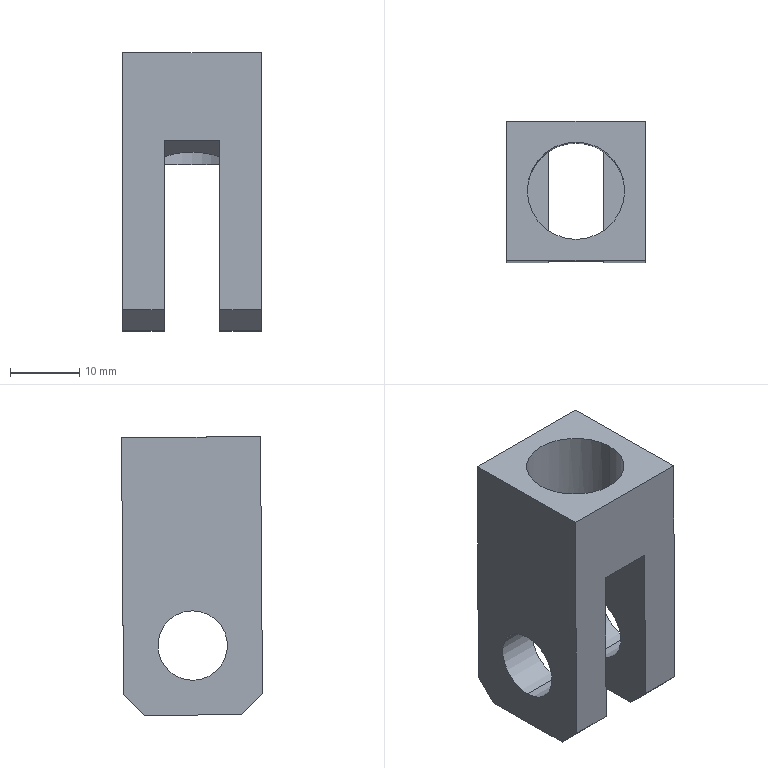Component | SolidWorks | OT-0100-008(LiveHinge)-1 | 1 solid | 23 faces | box 20 x 20.3 x 40.14 mm | volume 8582 mm3 | plane 17 | cylinder 6 | commonest cylinder face diameters 10 x4 14 x2 | material Plain Carbon Steel
build123d program:
from build123d import *

# Parameters (mm, degrees)
SKETCH1_W                  = 40
SKETCH1_H                  = 20
BOSS_EXTRUDE1_DEPTH        = 10
CUT_EXTRUDE1_REACH         = 47.826
SKETCH2_W                  = 24
SKETCH2_H                  = 8
M14X1_5_TAPPED_HOLE1_D     = 14
M14X1_5_TAPPED_HOLE1_DEPTH = 16
SKETCH5_R                  = 5
CUT_EXTRUDE2_DEPTH         = 46.826
CHAMFER1_SIZE              = 3
LUG_CLEARANCE_RELIEF_DEPTH = 4


with BuildPart() as part:
    # Sketch1 → Boss-Extrude1 (new, symmetric)
    with BuildSketch(Plane(origin=(0, 0, 0), x_dir=(1, 0, 0), z_dir=(0, 1, 0))):
        with Locations((20, 0)):
            Rectangle(SKETCH1_W, SKETCH1_H)
    extrude(amount=BOSS_EXTRUDE1_DEPTH, both=True)

    # Sketch2 → Cut-Extrude1 (cut, up to next)
    with BuildSketch(Plane(origin=(0, 10, 0), x_dir=(1, 0, 0), z_dir=(0, 1, 0)), mode=Mode.PRIVATE) as cut_extrude1_sk1:
        with Locations((12, 0)):
            Rectangle(SKETCH2_W, SKETCH2_H)
    cut_extrude1_tool1 = extrude(cut_extrude1_sk1.sketch, amount=-CUT_EXTRUDE1_REACH, mode=Mode.PRIVATE) & part.part
    add(cut_extrude1_tool1.solids().sort_by_distance((12, 10, 0))[0], mode=Mode.SUBTRACT)

    # M14x1.5 Tapped Hole1
    with Locations(Plane(origin=(40, 0, 0), x_dir=(0, 0, -1), z_dir=(1, 0, 0))):
        with Locations((0, 0)):
            Hole(M14X1_5_TAPPED_HOLE1_D / 2, depth=M14X1_5_TAPPED_HOLE1_DEPTH)

    # Sketch5 → Cut-Extrude2 (cut, through all)
    with BuildSketch(Plane.XY.offset(10)):
        with Locations((10, 0)):
            Circle(SKETCH5_R)
    extrude(amount=-CUT_EXTRUDE2_DEPTH, mode=Mode.SUBTRACT)

    # Chamfer1
    chamfer1_edges = [part.edges().sort_by_distance(p)[0] for p in [
        (0, -10, 7),
        (0, 10, 7),
        (0, 10, -7),
        (0, -10, -7),
    ]]
    chamfer(chamfer1_edges, length=CHAMFER1_SIZE)

    # Lug-clearance relief sketch → Lug-clearance relief (cut, symmetric)
    with BuildSketch(Plane.XY):
        Polygon((28.386, -12), (22, -0.1392), (22, -12), align=None)
    extrude(amount=LUG_CLEARANCE_RELIEF_DEPTH, both=True, mode=Mode.SUBTRACT)


solid = part.part

# Placed as in the assembly
solid = solid.moved(Location((200, 104.892, -36.996), (-0.4615, -90, 0)))
STEP:
#1=COLOUR_RGB('',0.7922,0.8196,0.9333);
#2=FILL_AREA_STYLE_COLOUR('',#1);
#3=FILL_AREA_STYLE('',(#2));
#4=SURFACE_STYLE_FILL_AREA(#3);
#5=SURFACE_SIDE_STYLE('',(#4));
#6=SURFACE_STYLE_USAGE(.BOTH.,#5);
#7=PRESENTATION_STYLE_ASSIGNMENT((#6));
#8=CARTESIAN_POINT('',(8.268,4.131,-1.26));
#9=VERTEX_POINT('',#8);
#10=CARTESIAN_POINT('',(8.268,4.134,-0.866));
#11=VERTEX_POINT('',#10);
#12=CARTESIAN_POINT('',(8.268,4.133,-1.063));
#13=DIRECTION('',(-1.,0.,-0.));
#14=DIRECTION('',(0.,0.008055,1.));
#15=AXIS2_PLACEMENT_3D('',#12,#13,#14);
#16=CIRCLE('',#15,0.1969);
#17=EDGE_CURVE('',#9,#11,#16,.T.);
#18=ORIENTED_EDGE('',*,*,#17,.F.);
#19=CARTESIAN_POINT('',(8.031,4.131,-1.26));
#20=VERTEX_POINT('',#19);
#21=CARTESIAN_POINT('',(8.268,4.131,-1.26));
#22=DIRECTION('',(-1.,0.,-0.));
#23=VECTOR('',#22,39.37);
#24=LINE('',#21,#23);
#25=EDGE_CURVE('',#9,#20,#24,.T.);
#26=ORIENTED_EDGE('',*,*,#25,.T.);
#27=CARTESIAN_POINT('',(8.031,4.134,-0.866));
#28=VERTEX_POINT('',#27);
#29=CARTESIAN_POINT('',(8.031,4.133,-1.063));
#30=DIRECTION('',(1.,-0.,0.));
#31=DIRECTION('',(0.,-0.008055,-1.));
#32=AXIS2_PLACEMENT_3D('',#29,#30,#31);
#33=CIRCLE('',#32,0.1969);
#34=EDGE_CURVE('',#28,#20,#33,.T.);
#35=ORIENTED_EDGE('',*,*,#34,.F.);
#36=CARTESIAN_POINT('',(8.268,4.134,-0.866));
#37=DIRECTION('',(-1.,0.,-0.));
#38=VECTOR('',#37,39.37);
#39=LINE('',#36,#38);
#40=EDGE_CURVE('',#11,#28,#39,.T.);
#41=ORIENTED_EDGE('',*,*,#40,.F.);
#42=EDGE_LOOP('',(#18,#26,#35,#41));
#43=FACE_OUTER_BOUND('',#42,.T.);
#44=CARTESIAN_POINT('',(8.268,4.133,-1.063));
#45=DIRECTION('',(-1.,0.,-0.));
#46=DIRECTION('',(0.,0.008055,1.));
#47=AXIS2_PLACEMENT_3D('',#44,#45,#46);
#48=CYLINDRICAL_SURFACE('',#47,0.1969);
#49=ADVANCED_FACE('',(#43),#48,.F.);
#50=CARTESIAN_POINT('',(7.717,4.131,-1.26));
#51=VERTEX_POINT('',#50);
#52=CARTESIAN_POINT('',(7.717,4.134,-0.866));
#53=VERTEX_POINT('',#52);
#54=CARTESIAN_POINT('',(7.717,4.133,-1.063));
#55=DIRECTION('',(-1.,0.,-0.));
#56=DIRECTION('',(0.,0.008055,1.));
#57=AXIS2_PLACEMENT_3D('',#54,#55,#56);
#58=CIRCLE('',#57,0.1969);
#59=EDGE_CURVE('',#51,#53,#58,.T.);
#60=ORIENTED_EDGE('',*,*,#59,.F.);
#61=CARTESIAN_POINT('',(7.48,4.131,-1.26));
#62=VERTEX_POINT('',#61);
#63=CARTESIAN_POINT('',(8.268,4.131,-1.26));
#64=DIRECTION('',(-1.,0.,-0.));
#65=VECTOR('',#64,39.37);
#66=LINE('',#63,#65);
#67=EDGE_CURVE('',#51,#62,#66,.T.);
#68=ORIENTED_EDGE('',*,*,#67,.T.);
#69=CARTESIAN_POINT('',(7.48,4.134,-0.866));
#70=VERTEX_POINT('',#69);
#71=CARTESIAN_POINT('',(7.48,4.133,-1.063));
#72=DIRECTION('',(-1.,0.,-0.));
#73=DIRECTION('',(0.,0.008055,1.));
#74=AXIS2_PLACEMENT_3D('',#71,#72,#73);
#75=CIRCLE('',#74,0.1969);
#76=EDGE_CURVE('',#62,#70,#75,.T.);
#77=ORIENTED_EDGE('',*,*,#76,.T.);
#78=CARTESIAN_POINT('',(8.268,4.134,-0.866));
#79=DIRECTION('',(-1.,0.,-0.));
#80=VECTOR('',#79,39.37);
#81=LINE('',#78,#80);
#82=EDGE_CURVE('',#53,#70,#81,.T.);
#83=ORIENTED_EDGE('',*,*,#82,.F.);
#84=EDGE_LOOP('',(#60,#68,#77,#83));
#85=FACE_OUTER_BOUND('',#84,.T.);
#86=CARTESIAN_POINT('',(8.268,4.133,-1.063));
#87=DIRECTION('',(-1.,0.,-0.));
#88=DIRECTION('',(0.,0.008055,1.));
#89=AXIS2_PLACEMENT_3D('',#86,#87,#88);
#90=CYLINDRICAL_SURFACE('',#89,0.1969);
#91=ADVANCED_FACE('',(#85),#90,.F.);
#92=CARTESIAN_POINT('',(7.717,3.911,-0.5098));
#93=VERTEX_POINT('',#92);
#94=CARTESIAN_POINT('',(7.598,4.137,-0.5117));
#95=VERTEX_POINT('',#94);
#96=CARTESIAN_POINT('',(7.874,4.137,-0.5117));
#97=DIRECTION('',(0.,-0.008055,-1.));
#98=DIRECTION('',(1.,0.,0.));
#99=AXIS2_PLACEMENT_3D('',#96,#97,#98);
#100=CIRCLE('',#99,0.2756);
#101=EDGE_CURVE('',#93,#95,#100,.T.);
#102=ORIENTED_EDGE('',*,*,#101,.T.);
#103=CARTESIAN_POINT('',(7.598,4.142,0.1182));
#104=VERTEX_POINT('',#103);
#105=CARTESIAN_POINT('',(7.598,4.142,0.1182));
#106=DIRECTION('',(-0.,0.008055,1.));
#107=VECTOR('',#106,39.37);
#108=LINE('',#105,#107);
#109=EDGE_CURVE('',#95,#104,#108,.T.);
#110=ORIENTED_EDGE('',*,*,#109,.T.);
#111=CARTESIAN_POINT('',(8.15,4.142,0.1182));
#112=VERTEX_POINT('',#111);
#113=CARTESIAN_POINT('',(7.874,4.142,0.1182));
#114=DIRECTION('',(-0.,0.008055,1.));
#115=DIRECTION('',(1.,0.,0.));
#116=AXIS2_PLACEMENT_3D('',#113,#114,#115);
#117=CIRCLE('',#116,0.2756);
#118=EDGE_CURVE('',#104,#112,#117,.T.);
#119=ORIENTED_EDGE('',*,*,#118,.T.);
#120=CARTESIAN_POINT('',(8.15,4.137,-0.5117));
#121=VERTEX_POINT('',#120);
#122=CARTESIAN_POINT('',(8.15,4.142,0.1182));
#123=DIRECTION('',(-0.,0.008055,1.));
#124=VECTOR('',#123,39.37);
#125=LINE('',#122,#124);
#126=EDGE_CURVE('',#121,#112,#125,.T.);
#127=ORIENTED_EDGE('',*,*,#126,.F.);
#128=CARTESIAN_POINT('',(8.031,3.911,-0.5098));
#129=VERTEX_POINT('',#128);
#130=CARTESIAN_POINT('',(7.874,4.137,-0.5117));
#131=DIRECTION('',(0.,-0.008055,-1.));
#132=DIRECTION('',(1.,0.,0.));
#133=AXIS2_PLACEMENT_3D('',#130,#131,#132);
#134=CIRCLE('',#133,0.2756);
#135=EDGE_CURVE('',#121,#129,#134,.T.);
#136=ORIENTED_EDGE('',*,*,#135,.T.);
#137=CARTESIAN_POINT('',(8.031,3.911,-0.4698));
#138=VERTEX_POINT('',#137);
#139=CARTESIAN_POINT('',(8.031,3.916,0.1201));
#140=DIRECTION('',(-0.,0.008055,1.));
#141=VECTOR('',#140,39.37);
#142=LINE('',#139,#141);
#143=EDGE_CURVE('',#129,#138,#142,.T.);
#144=ORIENTED_EDGE('',*,*,#143,.T.);
#145=CARTESIAN_POINT('',(7.717,3.911,-0.4698));
#146=VERTEX_POINT('',#145);
#147=CARTESIAN_POINT('',(8.031,3.911,-0.4698));
#148=CARTESIAN_POINT('',(7.934,3.844,-0.4325));
#149=CARTESIAN_POINT('',(7.814,3.844,-0.4325));
#150=CARTESIAN_POINT('',(7.717,3.911,-0.4698));
#151=(BOUNDED_CURVE()B_SPLINE_CURVE(3,(#147,#148,#149,#150),.UNSPECIFIED.,.F.,.F.)B_SPLINE_CURVE_WITH_KNOTS((4,4),(5.675,6.891),.UNSPECIFIED.)CURVE()GEOMETRIC_REPRESENTATION_ITEM()RATIONAL_B_SPLINE_CURVE((1.,0.8804,0.8804,1.))REPRESENTATION_ITEM(''));
#152=EDGE_CURVE('',#138,#146,#151,.T.);
#153=ORIENTED_EDGE('',*,*,#152,.T.);
#154=CARTESIAN_POINT('',(7.717,3.916,0.1201));
#155=DIRECTION('',(-0.,0.008055,1.));
#156=VECTOR('',#155,39.37);
#157=LINE('',#154,#156);
#158=EDGE_CURVE('',#93,#146,#157,.T.);
#159=ORIENTED_EDGE('',*,*,#158,.F.);
#160=EDGE_LOOP('',(#102,#110,#119,#127,#136,#144,#153,#159));
#161=FACE_OUTER_BOUND('',#160,.T.);
#162=CARTESIAN_POINT('',(7.874,4.142,0.1182));
#163=DIRECTION('',(-0.,0.008055,1.));
#164=DIRECTION('',(1.,0.,0.));
#165=AXIS2_PLACEMENT_3D('',#162,#163,#164);
#166=CYLINDRICAL_SURFACE('',#165,0.2756);
#167=ADVANCED_FACE('',(#161),#166,.F.);
#168=CARTESIAN_POINT('',(8.031,4.363,-0.5135));
#169=VERTEX_POINT('',#168);
#170=CARTESIAN_POINT('',(8.031,4.531,-0.5148));
#171=VERTEX_POINT('',#170);
#172=CARTESIAN_POINT('',(8.031,3.744,-0.5085));
#173=DIRECTION('',(0.,1.,-0.008055));
#174=VECTOR('',#173,39.37);
#175=LINE('',#172,#174);
#176=EDGE_CURVE('',#169,#171,#175,.T.);
#177=ORIENTED_EDGE('',*,*,#176,.F.);
#178=CARTESIAN_POINT('',(7.717,4.363,-0.5135));
#179=VERTEX_POINT('',#178);
#180=CARTESIAN_POINT('',(7.874,4.137,-0.5117));
#181=DIRECTION('',(-0.,0.008055,1.));
#182=DIRECTION('',(1.,0.,0.));
#183=AXIS2_PLACEMENT_3D('',#180,#181,#182);
#184=CIRCLE('',#183,0.2756);
#185=EDGE_CURVE('',#169,#179,#184,.T.);
#186=ORIENTED_EDGE('',*,*,#185,.T.);
#187=CARTESIAN_POINT('',(7.717,4.531,-0.5148));
#188=VERTEX_POINT('',#187);
#189=CARTESIAN_POINT('',(7.717,3.744,-0.5085));
#190=DIRECTION('',(0.,1.,-0.008055));
#191=VECTOR('',#190,39.37);
#192=LINE('',#189,#191);
#193=EDGE_CURVE('',#179,#188,#192,.T.);
#194=ORIENTED_EDGE('',*,*,#193,.T.);
#195=CARTESIAN_POINT('',(7.717,4.531,-0.5148));
#196=DIRECTION('',(1.,-0.,0.));
#197=VECTOR('',#196,39.37);
#198=LINE('',#195,#197);
#199=EDGE_CURVE('',#188,#171,#198,.T.);
#200=ORIENTED_EDGE('',*,*,#199,.T.);
#201=EDGE_LOOP('',(#177,#186,#194,#200));
#202=FACE_OUTER_BOUND('',#201,.T.);
#203=CARTESIAN_POINT('',(7.717,3.744,-0.5085));
#204=DIRECTION('',(-0.,0.008055,1.));
#205=DIRECTION('',(1.,-0.,0.));
#206=AXIS2_PLACEMENT_3D('',#203,#204,#205);
#207=PLANE('',#206);
#208=ADVANCED_FACE('',(#202),#207,.F.);
#209=CARTESIAN_POINT('',(8.268,4.405,-1.459));
#210=VERTEX_POINT('',#209);
#211=CARTESIAN_POINT('',(8.268,3.854,-1.454));
#212=VERTEX_POINT('',#211);
#213=CARTESIAN_POINT('',(8.268,4.523,-1.46));
#214=DIRECTION('',(-0.,-1.,0.008055));
#215=VECTOR('',#214,39.37);
#216=LINE('',#213,#215);
#217=EDGE_CURVE('',#210,#212,#216,.T.);
#218=ORIENTED_EDGE('',*,*,#217,.T.);
#219=CARTESIAN_POINT('',(8.031,3.854,-1.454));
#220=VERTEX_POINT('',#219);
#221=CARTESIAN_POINT('',(8.031,3.854,-1.454));
#222=DIRECTION('',(-1.,0.,-0.));
#223=VECTOR('',#222,39.37);
#224=LINE('',#221,#223);
#225=EDGE_CURVE('',#212,#220,#224,.T.);
#226=ORIENTED_EDGE('',*,*,#225,.T.);
#227=CARTESIAN_POINT('',(8.031,4.405,-1.459));
#228=VERTEX_POINT('',#227);
#229=CARTESIAN_POINT('',(8.031,3.736,-1.453));
#230=DIRECTION('',(0.,1.,-0.008055));
#231=VECTOR('',#230,39.37);
#232=LINE('',#229,#231);
#233=EDGE_CURVE('',#220,#228,#232,.T.);
#234=ORIENTED_EDGE('',*,*,#233,.T.);
#235=CARTESIAN_POINT('',(7.48,4.405,-1.459));
#236=DIRECTION('',(1.,-0.,0.));
#237=VECTOR('',#236,39.37);
#238=LINE('',#235,#237);
#239=EDGE_CURVE('',#228,#210,#238,.T.);
#240=ORIENTED_EDGE('',*,*,#239,.T.);
#241=EDGE_LOOP('',(#218,#226,#234,#240));
#242=FACE_OUTER_BOUND('',#241,.T.);
#243=CARTESIAN_POINT('',(7.48,4.523,-1.46));
#244=DIRECTION('',(-0.,0.008055,1.));
#245=DIRECTION('',(1.,-0.,0.));
#246=AXIS2_PLACEMENT_3D('',#243,#244,#245);
#247=PLANE('',#246);
#248=ADVANCED_FACE('',(#242),#247,.F.);
#249=CARTESIAN_POINT('',(7.717,3.854,-1.454));
#250=VERTEX_POINT('',#249);
#251=CARTESIAN_POINT('',(7.717,4.405,-1.459));
#252=VERTEX_POINT('',#251);
#253=CARTESIAN_POINT('',(7.717,3.736,-1.453));
#254=DIRECTION('',(0.,1.,-0.008055));
#255=VECTOR('',#254,39.37);
#256=LINE('',#253,#255);
#257=EDGE_CURVE('',#250,#252,#256,.T.);
#258=ORIENTED_EDGE('',*,*,#257,.F.);
#259=CARTESIAN_POINT('',(7.48,3.854,-1.454));
#260=VERTEX_POINT('',#259);
#261=CARTESIAN_POINT('',(7.48,3.854,-1.454));
#262=DIRECTION('',(-1.,0.,-0.));
#263=VECTOR('',#262,39.37);
#264=LINE('',#261,#263);
#265=EDGE_CURVE('',#250,#260,#264,.T.);
#266=ORIENTED_EDGE('',*,*,#265,.T.);
#267=CARTESIAN_POINT('',(7.48,4.405,-1.459));
#268=VERTEX_POINT('',#267);
#269=CARTESIAN_POINT('',(7.48,4.523,-1.46));
#270=DIRECTION('',(-0.,-1.,0.008055));
#271=VECTOR('',#270,39.37);
#272=LINE('',#269,#271);
#273=EDGE_CURVE('',#268,#260,#272,.T.);
#274=ORIENTED_EDGE('',*,*,#273,.F.);
#275=CARTESIAN_POINT('',(7.48,4.405,-1.459));
#276=DIRECTION('',(1.,-0.,0.));
#277=VECTOR('',#276,39.37);
#278=LINE('',#275,#277);
#279=EDGE_CURVE('',#268,#252,#278,.T.);
#280=ORIENTED_EDGE('',*,*,#279,.T.);
#281=EDGE_LOOP('',(#258,#266,#274,#280));
#282=FACE_OUTER_BOUND('',#281,.T.);
#283=CARTESIAN_POINT('',(7.48,4.523,-1.46));
#284=DIRECTION('',(-0.,0.008055,1.));
#285=DIRECTION('',(1.,-0.,0.));
#286=AXIS2_PLACEMENT_3D('',#283,#284,#285);
#287=PLANE('',#286);
#288=ADVANCED_FACE('',(#282),#287,.F.);
#289=CARTESIAN_POINT('',(7.48,4.133,-1.063));
#290=DIRECTION('',(-1.,0.,-0.));
#291=DIRECTION('',(0.,0.008055,1.));
#292=AXIS2_PLACEMENT_3D('',#289,#290,#291);
#293=CIRCLE('',#292,0.1969);
#294=EDGE_CURVE('',#70,#62,#293,.T.);
#295=ORIENTED_EDGE('',*,*,#294,.F.);
#296=ORIENTED_EDGE('',*,*,#76,.F.);
#297=EDGE_LOOP('',(#295,#296));
#298=FACE_BOUND('',#297,.T.);
#299=ORIENTED_EDGE('',*,*,#273,.T.);
#300=CARTESIAN_POINT('',(7.48,3.737,-1.335));
#301=VERTEX_POINT('',#300);
#302=CARTESIAN_POINT('',(7.48,3.854,-1.454));
#303=DIRECTION('',(-0.,-0.7014,0.7128));
#304=VECTOR('',#303,39.37);
#305=LINE('',#302,#304);
#306=EDGE_CURVE('',#260,#301,#305,.T.);
#307=ORIENTED_EDGE('',*,*,#306,.T.);
#308=CARTESIAN_POINT('',(7.48,3.749,0.1214));
#309=VERTEX_POINT('',#308);
#310=CARTESIAN_POINT('',(7.48,3.736,-1.453));
#311=DIRECTION('',(-0.,0.008055,1.));
#312=VECTOR('',#311,39.37);
#313=LINE('',#310,#312);
#314=EDGE_CURVE('',#301,#309,#313,.T.);
#315=ORIENTED_EDGE('',*,*,#314,.T.);
#316=CARTESIAN_POINT('',(7.48,4.536,0.1151));
#317=VERTEX_POINT('',#316);
#318=CARTESIAN_POINT('',(7.48,4.536,0.1151));
#319=DIRECTION('',(-0.,-1.,0.008055));
#320=VECTOR('',#319,39.37);
#321=LINE('',#318,#320);
#322=EDGE_CURVE('',#317,#309,#321,.T.);
#323=ORIENTED_EDGE('',*,*,#322,.F.);
#324=CARTESIAN_POINT('',(7.48,4.524,-1.342));
#325=VERTEX_POINT('',#324);
#326=CARTESIAN_POINT('',(7.48,4.523,-1.46));
#327=DIRECTION('',(-0.,0.008055,1.));
#328=VECTOR('',#327,39.37);
#329=LINE('',#326,#328);
#330=EDGE_CURVE('',#325,#317,#329,.T.);
#331=ORIENTED_EDGE('',*,*,#330,.F.);
#332=CARTESIAN_POINT('',(7.48,4.524,-1.342));
#333=DIRECTION('',(-0.,-0.7128,-0.7014));
#334=VECTOR('',#333,39.37);
#335=LINE('',#332,#334);
#336=EDGE_CURVE('',#325,#268,#335,.T.);
#337=ORIENTED_EDGE('',*,*,#336,.T.);
#338=EDGE_LOOP('',(#299,#307,#315,#323,#331,#337));
#339=FACE_OUTER_BOUND('',#338,.T.);
#340=CARTESIAN_POINT('',(7.48,4.523,-1.46));
#341=DIRECTION('',(1.,-0.,0.));
#342=DIRECTION('',(0.,-0.008055,-1.));
#343=AXIS2_PLACEMENT_3D('',#340,#341,#342);
#344=PLANE('',#343);
#345=ADVANCED_FACE('',(#298,#339),#344,.F.);
#346=CARTESIAN_POINT('',(7.874,4.142,0.1182));
#347=DIRECTION('',(-0.,0.008055,1.));
#348=DIRECTION('',(1.,0.,0.));
#349=AXIS2_PLACEMENT_3D('',#346,#347,#348);
#350=CIRCLE('',#349,0.2756);
#351=EDGE_CURVE('',#112,#104,#350,.T.);
#352=ORIENTED_EDGE('',*,*,#351,.F.);
#353=ORIENTED_EDGE('',*,*,#118,.F.);
#354=EDGE_LOOP('',(#352,#353));
#355=FACE_BOUND('',#354,.T.);
#356=CARTESIAN_POINT('',(8.268,3.749,0.1214));
#357=VERTEX_POINT('',#356);
#358=CARTESIAN_POINT('',(7.48,3.749,0.1214));
#359=DIRECTION('',(1.,-0.,0.));
#360=VECTOR('',#359,39.37);
#361=LINE('',#358,#360);
#362=EDGE_CURVE('',#309,#357,#361,.T.);
#363=ORIENTED_EDGE('',*,*,#362,.T.);
#364=CARTESIAN_POINT('',(8.268,4.536,0.1151));
#365=VERTEX_POINT('',#364);
#366=CARTESIAN_POINT('',(8.268,4.536,0.1151));
#367=DIRECTION('',(-0.,-1.,0.008055));
#368=VECTOR('',#367,39.37);
#369=LINE('',#366,#368);
#370=EDGE_CURVE('',#365,#357,#369,.T.);
#371=ORIENTED_EDGE('',*,*,#370,.F.);
#372=CARTESIAN_POINT('',(7.48,4.536,0.1151));
#373=DIRECTION('',(1.,-0.,0.));
#374=VECTOR('',#373,39.37);
#375=LINE('',#372,#374);
#376=EDGE_CURVE('',#317,#365,#375,.T.);
#377=ORIENTED_EDGE('',*,*,#376,.F.);
#378=ORIENTED_EDGE('',*,*,#322,.T.);
#379=EDGE_LOOP('',(#363,#371,#377,#378));
#380=FACE_OUTER_BOUND('',#379,.T.);
#381=CARTESIAN_POINT('',(7.48,4.536,0.1151));
#382=DIRECTION('',(0.,-0.008055,-1.));
#383=DIRECTION('',(-1.,0.,-0.));
#384=AXIS2_PLACEMENT_3D('',#381,#382,#383);
#385=PLANE('',#384);
#386=ADVANCED_FACE('',(#355,#380),#385,.F.);
#387=CARTESIAN_POINT('',(8.268,4.133,-1.063));
#388=DIRECTION('',(-1.,0.,-0.));
#389=DIRECTION('',(0.,0.008055,1.));
#390=AXIS2_PLACEMENT_3D('',#387,#388,#389);
#391=CIRCLE('',#390,0.1969);
#392=EDGE_CURVE('',#11,#9,#391,.T.);
#393=ORIENTED_EDGE('',*,*,#392,.T.);
#394=ORIENTED_EDGE('',*,*,#17,.T.);
#395=EDGE_LOOP('',(#393,#394));
#396=FACE_BOUND('',#395,.T.);
#397=CARTESIAN_POINT('',(8.268,3.737,-1.335));
#398=VERTEX_POINT('',#397);
#399=CARTESIAN_POINT('',(8.268,3.736,-1.453));
#400=DIRECTION('',(-0.,-0.008055,-1.));
#401=VECTOR('',#400,39.37);
#402=LINE('',#399,#401);
#403=EDGE_CURVE('',#357,#398,#402,.T.);
#404=ORIENTED_EDGE('',*,*,#403,.T.);
#405=CARTESIAN_POINT('',(8.268,3.854,-1.454));
#406=DIRECTION('',(-0.,0.7014,-0.7128));
#407=VECTOR('',#406,39.37);
#408=LINE('',#405,#407);
#409=EDGE_CURVE('',#398,#212,#408,.T.);
#410=ORIENTED_EDGE('',*,*,#409,.T.);
#411=ORIENTED_EDGE('',*,*,#217,.F.);
#412=CARTESIAN_POINT('',(8.268,4.524,-1.342));
#413=VERTEX_POINT('',#412);
#414=CARTESIAN_POINT('',(8.268,4.524,-1.342));
#415=DIRECTION('',(0.,0.7128,0.7014));
#416=VECTOR('',#415,39.37);
#417=LINE('',#414,#416);
#418=EDGE_CURVE('',#210,#413,#417,.T.);
#419=ORIENTED_EDGE('',*,*,#418,.T.);
#420=CARTESIAN_POINT('',(8.268,4.523,-1.46));
#421=DIRECTION('',(-0.,-0.008055,-1.));
#422=VECTOR('',#421,39.37);
#423=LINE('',#420,#422);
#424=EDGE_CURVE('',#365,#413,#423,.T.);
#425=ORIENTED_EDGE('',*,*,#424,.F.);
#426=ORIENTED_EDGE('',*,*,#370,.T.);
#427=EDGE_LOOP('',(#404,#410,#411,#419,#425,#426));
#428=FACE_OUTER_BOUND('',#427,.T.);
#429=CARTESIAN_POINT('',(8.268,4.523,-1.46));
#430=DIRECTION('',(-1.,0.,0.));
#431=DIRECTION('',(0.,0.008055,1.));
#432=AXIS2_PLACEMENT_3D('',#429,#430,#431);
#433=PLANE('',#432);
#434=ADVANCED_FACE('',(#396,#428),#433,.F.);
#435=ORIENTED_EDGE('',*,*,#424,.T.);
#436=CARTESIAN_POINT('',(8.031,4.524,-1.342));
#437=VERTEX_POINT('',#436);
#438=CARTESIAN_POINT('',(7.874,4.524,-1.342));
#439=DIRECTION('',(-1.,0.,-0.));
#440=VECTOR('',#439,39.37);
#441=LINE('',#438,#440);
#442=EDGE_CURVE('',#413,#437,#441,.T.);
#443=ORIENTED_EDGE('',*,*,#442,.T.);
#444=CARTESIAN_POINT('',(8.031,4.523,-1.46));
#445=DIRECTION('',(0.,-0.008055,-1.));
#446=VECTOR('',#445,39.37);
#447=LINE('',#444,#446);
#448=EDGE_CURVE('',#171,#437,#447,.T.);
#449=ORIENTED_EDGE('',*,*,#448,.F.);
#450=ORIENTED_EDGE('',*,*,#199,.F.);
#451=CARTESIAN_POINT('',(7.717,4.524,-1.342));
#452=VERTEX_POINT('',#451);
#453=CARTESIAN_POINT('',(7.717,4.523,-1.46));
#454=DIRECTION('',(-0.,0.008055,1.));
#455=VECTOR('',#454,39.37);
#456=LINE('',#453,#455);
#457=EDGE_CURVE('',#452,#188,#456,.T.);
#458=ORIENTED_EDGE('',*,*,#457,.F.);
#459=CARTESIAN_POINT('',(7.874,4.524,-1.342));
#460=DIRECTION('',(-1.,0.,-0.));
#461=VECTOR('',#460,39.37);
#462=LINE('',#459,#461);
#463=EDGE_CURVE('',#452,#325,#462,.T.);
#464=ORIENTED_EDGE('',*,*,#463,.T.);
#465=ORIENTED_EDGE('',*,*,#330,.T.);
#466=ORIENTED_EDGE('',*,*,#376,.T.);
#467=EDGE_LOOP('',(#435,#443,#449,#450,#458,#464,#465,#466));
#468=FACE_OUTER_BOUND('',#467,.T.);
#469=CARTESIAN_POINT('',(7.874,4.523,-1.46));
#470=DIRECTION('',(-0.,-1.,0.008055));
#471=DIRECTION('',(1.,-0.,0.));
#472=AXIS2_PLACEMENT_3D('',#469,#470,#471);
#473=PLANE('',#472);
#474=ADVANCED_FACE('',(#468),#473,.F.);
#475=CARTESIAN_POINT('',(8.031,3.745,-0.3782));
#476=VERTEX_POINT('',#475);
#477=CARTESIAN_POINT('',(7.717,3.745,-0.3782));
#478=VERTEX_POINT('',#477);
#479=CARTESIAN_POINT('',(7.874,3.745,-0.3782));
#480=DIRECTION('',(-1.,0.,-0.));
#481=VECTOR('',#480,39.37);
#482=LINE('',#479,#481);
#483=EDGE_CURVE('',#476,#478,#482,.T.);
#484=ORIENTED_EDGE('',*,*,#483,.F.);
#485=CARTESIAN_POINT('',(8.031,3.737,-1.335));
#486=VERTEX_POINT('',#485);
#487=CARTESIAN_POINT('',(8.031,3.736,-1.453));
#488=DIRECTION('',(0.,-0.008055,-1.));
#489=VECTOR('',#488,39.37);
#490=LINE('',#487,#489);
#491=EDGE_CURVE('',#476,#486,#490,.T.);
#492=ORIENTED_EDGE('',*,*,#491,.T.);
#493=CARTESIAN_POINT('',(8.268,3.737,-1.335));
#494=DIRECTION('',(1.,-0.,0.));
#495=VECTOR('',#494,39.37);
#496=LINE('',#493,#495);
#497=EDGE_CURVE('',#486,#398,#496,.T.);
#498=ORIENTED_EDGE('',*,*,#497,.T.);
#499=ORIENTED_EDGE('',*,*,#403,.F.);
#500=ORIENTED_EDGE('',*,*,#362,.F.);
#501=ORIENTED_EDGE('',*,*,#314,.F.);
#502=CARTESIAN_POINT('',(7.717,3.737,-1.335));
#503=VERTEX_POINT('',#502);
#504=CARTESIAN_POINT('',(7.717,3.737,-1.335));
#505=DIRECTION('',(1.,-0.,0.));
#506=VECTOR('',#505,39.37);
#507=LINE('',#504,#506);
#508=EDGE_CURVE('',#301,#503,#507,.T.);
#509=ORIENTED_EDGE('',*,*,#508,.T.);
#510=CARTESIAN_POINT('',(7.717,3.736,-1.453));
#511=DIRECTION('',(-0.,0.008055,1.));
#512=VECTOR('',#511,39.37);
#513=LINE('',#510,#512);
#514=EDGE_CURVE('',#503,#478,#513,.T.);
#515=ORIENTED_EDGE('',*,*,#514,.T.);
#516=EDGE_LOOP('',(#484,#492,#498,#499,#500,#501,#509,#515));
#517=FACE_OUTER_BOUND('',#516,.T.);
#518=CARTESIAN_POINT('',(7.874,3.736,-1.453));
#519=DIRECTION('',(-0.,-1.,0.008055));
#520=DIRECTION('',(1.,-0.,0.));
#521=AXIS2_PLACEMENT_3D('',#518,#519,#520);
#522=PLANE('',#521);
#523=ADVANCED_FACE('',(#517),#522,.T.);
#524=CARTESIAN_POINT('',(8.031,3.854,-1.454));
#525=DIRECTION('',(-0.,-0.7014,0.7128));
#526=VECTOR('',#525,39.37);
#527=LINE('',#524,#526);
#528=EDGE_CURVE('',#220,#486,#527,.T.);
#529=ORIENTED_EDGE('',*,*,#528,.T.);
#530=ORIENTED_EDGE('',*,*,#491,.F.);
#531=CARTESIAN_POINT('',(8.031,3.666,-0.3352));
#532=DIRECTION('',(0.,0.8767,-0.4811));
#533=VECTOR('',#532,39.37);
#534=LINE('',#531,#533);
#535=EDGE_CURVE('',#476,#138,#534,.T.);
#536=ORIENTED_EDGE('',*,*,#535,.T.);
#537=ORIENTED_EDGE('',*,*,#143,.F.);
#538=CARTESIAN_POINT('',(8.031,3.744,-0.5085));
#539=DIRECTION('',(0.,1.,-0.008055));
#540=VECTOR('',#539,39.37);
#541=LINE('',#538,#540);
#542=EDGE_CURVE('',#129,#169,#541,.T.);
#543=ORIENTED_EDGE('',*,*,#542,.T.);
#544=ORIENTED_EDGE('',*,*,#176,.T.);
#545=ORIENTED_EDGE('',*,*,#448,.T.);
#546=CARTESIAN_POINT('',(8.031,4.524,-1.342));
#547=DIRECTION('',(-0.,-0.7128,-0.7014));
#548=VECTOR('',#547,39.37);
#549=LINE('',#546,#548);
#550=EDGE_CURVE('',#437,#228,#549,.T.);
#551=ORIENTED_EDGE('',*,*,#550,.T.);
#552=ORIENTED_EDGE('',*,*,#233,.F.);
#553=EDGE_LOOP('',(#529,#530,#536,#537,#543,#544,#545,#551,#552));
#554=FACE_OUTER_BOUND('',#553,.T.);
#555=ORIENTED_EDGE('',*,*,#34,.T.);
#556=CARTESIAN_POINT('',(8.031,4.133,-1.063));
#557=DIRECTION('',(1.,-0.,0.));
#558=DIRECTION('',(0.,-0.008055,-1.));
#559=AXIS2_PLACEMENT_3D('',#556,#557,#558);
#560=CIRCLE('',#559,0.1969);
#561=EDGE_CURVE('',#20,#28,#560,.T.);
#562=ORIENTED_EDGE('',*,*,#561,.T.);
#563=EDGE_LOOP('',(#555,#562));
#564=FACE_BOUND('',#563,.T.);
#565=CARTESIAN_POINT('',(8.031,3.736,-1.453));
#566=DIRECTION('',(1.,-0.,0.));
#567=DIRECTION('',(0.,-0.008055,-1.));
#568=AXIS2_PLACEMENT_3D('',#565,#566,#567);
#569=PLANE('',#568);
#570=ADVANCED_FACE('',(#554,#564),#569,.F.);
#571=CARTESIAN_POINT('',(7.717,4.133,-1.063));
#572=DIRECTION('',(-1.,0.,-0.));
#573=DIRECTION('',(0.,0.008055,1.));
#574=AXIS2_PLACEMENT_3D('',#571,#572,#573);
#575=CIRCLE('',#574,0.1969);
#576=EDGE_CURVE('',#53,#51,#575,.T.);
#577=ORIENTED_EDGE('',*,*,#576,.T.);
#578=ORIENTED_EDGE('',*,*,#59,.T.);
#579=EDGE_LOOP('',(#577,#578));
#580=FACE_BOUND('',#579,.T.);
#581=ORIENTED_EDGE('',*,*,#193,.F.);
#582=CARTESIAN_POINT('',(7.717,3.744,-0.5085));
#583=DIRECTION('',(0.,1.,-0.008055));
#584=VECTOR('',#583,39.37);
#585=LINE('',#582,#584);
#586=EDGE_CURVE('',#93,#179,#585,.T.);
#587=ORIENTED_EDGE('',*,*,#586,.F.);
#588=ORIENTED_EDGE('',*,*,#158,.T.);
#589=CARTESIAN_POINT('',(7.717,3.666,-0.3352));
#590=DIRECTION('',(0.,0.8767,-0.4811));
#591=VECTOR('',#590,39.37);
#592=LINE('',#589,#591);
#593=EDGE_CURVE('',#478,#146,#592,.T.);
#594=ORIENTED_EDGE('',*,*,#593,.F.);
#595=ORIENTED_EDGE('',*,*,#514,.F.);
#596=CARTESIAN_POINT('',(7.717,3.854,-1.454));
#597=DIRECTION('',(0.,0.7014,-0.7128));
#598=VECTOR('',#597,39.37);
#599=LINE('',#596,#598);
#600=EDGE_CURVE('',#503,#250,#599,.T.);
#601=ORIENTED_EDGE('',*,*,#600,.T.);
#602=ORIENTED_EDGE('',*,*,#257,.T.);
#603=CARTESIAN_POINT('',(7.717,4.524,-1.342));
#604=DIRECTION('',(0.,0.7128,0.7014));
#605=VECTOR('',#604,39.37);
#606=LINE('',#603,#605);
#607=EDGE_CURVE('',#252,#452,#606,.T.);
#608=ORIENTED_EDGE('',*,*,#607,.T.);
#609=ORIENTED_EDGE('',*,*,#457,.T.);
#610=EDGE_LOOP('',(#581,#587,#588,#594,#595,#601,#602,#608,#609));
#611=FACE_OUTER_BOUND('',#610,.T.);
#612=CARTESIAN_POINT('',(7.717,3.736,-1.453));
#613=DIRECTION('',(-1.,0.,-0.));
#614=DIRECTION('',(-0.,0.008055,1.));
#615=AXIS2_PLACEMENT_3D('',#612,#613,#614);
#616=PLANE('',#615);
#617=ADVANCED_FACE('',(#580,#611),#616,.F.);
#618=ORIENTED_EDGE('',*,*,#586,.T.);
#619=CARTESIAN_POINT('',(7.874,4.137,-0.5117));
#620=DIRECTION('',(0.,-0.008055,-1.));
#621=DIRECTION('',(1.,0.,0.));
#622=AXIS2_PLACEMENT_3D('',#619,#620,#621);
#623=CIRCLE('',#622,0.2756);
#624=EDGE_CURVE('',#95,#179,#623,.T.);
#625=ORIENTED_EDGE('',*,*,#624,.F.);
#626=ORIENTED_EDGE('',*,*,#101,.F.);
#627=EDGE_LOOP('',(#618,#625,#626));
#628=FACE_OUTER_BOUND('',#627,.T.);
#629=CARTESIAN_POINT('',(7.717,3.744,-0.5085));
#630=DIRECTION('',(-0.,0.008055,1.));
#631=DIRECTION('',(1.,-0.,0.));
#632=AXIS2_PLACEMENT_3D('',#629,#630,#631);
#633=PLANE('',#632);
#634=ADVANCED_FACE('',(#628),#633,.T.);
#635=ORIENTED_EDGE('',*,*,#109,.F.);
#636=ORIENTED_EDGE('',*,*,#624,.T.);
#637=ORIENTED_EDGE('',*,*,#185,.F.);
#638=CARTESIAN_POINT('',(7.874,4.137,-0.5117));
#639=DIRECTION('',(0.,-0.008055,-1.));
#640=DIRECTION('',(1.,0.,0.));
#641=AXIS2_PLACEMENT_3D('',#638,#639,#640);
#642=CIRCLE('',#641,0.2756);
#643=EDGE_CURVE('',#169,#121,#642,.T.);
#644=ORIENTED_EDGE('',*,*,#643,.T.);
#645=ORIENTED_EDGE('',*,*,#126,.T.);
#646=ORIENTED_EDGE('',*,*,#351,.T.);
#647=EDGE_LOOP('',(#635,#636,#637,#644,#645,#646));
#648=FACE_OUTER_BOUND('',#647,.T.);
#649=CARTESIAN_POINT('',(7.874,4.142,0.1182));
#650=DIRECTION('',(-0.,0.008055,1.));
#651=DIRECTION('',(1.,0.,0.));
#652=AXIS2_PLACEMENT_3D('',#649,#650,#651);
#653=CYLINDRICAL_SURFACE('',#652,0.2756);
#654=ADVANCED_FACE('',(#648),#653,.F.);
#655=ORIENTED_EDGE('',*,*,#643,.F.);
#656=ORIENTED_EDGE('',*,*,#542,.F.);
#657=ORIENTED_EDGE('',*,*,#135,.F.);
#658=EDGE_LOOP('',(#655,#656,#657));
#659=FACE_OUTER_BOUND('',#658,.T.);
#660=CARTESIAN_POINT('',(7.717,3.744,-0.5085));
#661=DIRECTION('',(-0.,0.008055,1.));
#662=DIRECTION('',(1.,-0.,0.));
#663=AXIS2_PLACEMENT_3D('',#660,#661,#662);
#664=PLANE('',#663);
#665=ADVANCED_FACE('',(#659),#664,.T.);
#666=ORIENTED_EDGE('',*,*,#67,.F.);
#667=ORIENTED_EDGE('',*,*,#576,.F.);
#668=ORIENTED_EDGE('',*,*,#82,.T.);
#669=ORIENTED_EDGE('',*,*,#294,.T.);
#670=EDGE_LOOP('',(#666,#667,#668,#669));
#671=FACE_OUTER_BOUND('',#670,.T.);
#672=CARTESIAN_POINT('',(8.268,4.133,-1.063));
#673=DIRECTION('',(-1.,0.,-0.));
#674=DIRECTION('',(0.,0.008055,1.));
#675=AXIS2_PLACEMENT_3D('',#672,#673,#674);
#676=CYLINDRICAL_SURFACE('',#675,0.1969);
#677=ADVANCED_FACE('',(#671),#676,.F.);
#678=ORIENTED_EDGE('',*,*,#25,.F.);
#679=ORIENTED_EDGE('',*,*,#392,.F.);
#680=ORIENTED_EDGE('',*,*,#40,.T.);
#681=ORIENTED_EDGE('',*,*,#561,.F.);
#682=EDGE_LOOP('',(#678,#679,#680,#681));
#683=FACE_OUTER_BOUND('',#682,.T.);
#684=CARTESIAN_POINT('',(8.268,4.133,-1.063));
#685=DIRECTION('',(-1.,0.,-0.));
#686=DIRECTION('',(0.,0.008055,1.));
#687=AXIS2_PLACEMENT_3D('',#684,#685,#686);
#688=CYLINDRICAL_SURFACE('',#687,0.1969);
#689=ADVANCED_FACE('',(#683),#688,.F.);
#690=ORIENTED_EDGE('',*,*,#409,.F.);
#691=ORIENTED_EDGE('',*,*,#497,.F.);
#692=ORIENTED_EDGE('',*,*,#528,.F.);
#693=ORIENTED_EDGE('',*,*,#225,.F.);
#694=EDGE_LOOP('',(#690,#691,#692,#693));
#695=FACE_OUTER_BOUND('',#694,.T.);
#696=CARTESIAN_POINT('',(7.48,3.854,-1.454));
#697=DIRECTION('',(-0.,-0.7128,-0.7014));
#698=DIRECTION('',(1.,-0.,0.));
#699=AXIS2_PLACEMENT_3D('',#696,#697,#698);
#700=PLANE('',#699);
#701=ADVANCED_FACE('',(#695),#700,.T.);
#702=ORIENTED_EDGE('',*,*,#600,.F.);
#703=ORIENTED_EDGE('',*,*,#508,.F.);
#704=ORIENTED_EDGE('',*,*,#306,.F.);
#705=ORIENTED_EDGE('',*,*,#265,.F.);
#706=EDGE_LOOP('',(#702,#703,#704,#705));
#707=FACE_OUTER_BOUND('',#706,.T.);
#708=CARTESIAN_POINT('',(7.48,3.854,-1.454));
#709=DIRECTION('',(-0.,-0.7128,-0.7014));
#710=DIRECTION('',(1.,-0.,0.));
#711=AXIS2_PLACEMENT_3D('',#708,#709,#710);
#712=PLANE('',#711);
#713=ADVANCED_FACE('',(#707),#712,.T.);
#714=ORIENTED_EDGE('',*,*,#418,.F.);
#715=ORIENTED_EDGE('',*,*,#239,.F.);
#716=ORIENTED_EDGE('',*,*,#550,.F.);
#717=ORIENTED_EDGE('',*,*,#442,.F.);
#718=EDGE_LOOP('',(#714,#715,#716,#717));
#719=FACE_OUTER_BOUND('',#718,.T.);
#720=CARTESIAN_POINT('',(7.874,4.524,-1.342));
#721=DIRECTION('',(-0.,-0.7014,0.7128));
#722=DIRECTION('',(-1.,0.,-0.));
#723=AXIS2_PLACEMENT_3D('',#720,#721,#722);
#724=PLANE('',#723);
#725=ADVANCED_FACE('',(#719),#724,.F.);
#726=ORIENTED_EDGE('',*,*,#607,.F.);
#727=ORIENTED_EDGE('',*,*,#279,.F.);
#728=ORIENTED_EDGE('',*,*,#336,.F.);
#729=ORIENTED_EDGE('',*,*,#463,.F.);
#730=EDGE_LOOP('',(#726,#727,#728,#729));
#731=FACE_OUTER_BOUND('',#730,.T.);
#732=CARTESIAN_POINT('',(7.874,4.524,-1.342));
#733=DIRECTION('',(-0.,-0.7014,0.7128));
#734=DIRECTION('',(-1.,0.,-0.));
#735=AXIS2_PLACEMENT_3D('',#732,#733,#734);
#736=PLANE('',#735);
#737=ADVANCED_FACE('',(#731),#736,.F.);
#738=ORIENTED_EDGE('',*,*,#483,.T.);
#739=ORIENTED_EDGE('',*,*,#593,.T.);
#740=ORIENTED_EDGE('',*,*,#152,.F.);
#741=ORIENTED_EDGE('',*,*,#535,.F.);
#742=EDGE_LOOP('',(#738,#739,#740,#741));
#743=FACE_OUTER_BOUND('',#742,.T.);
#744=CARTESIAN_POINT('',(8.031,3.666,-0.3352));
#745=DIRECTION('',(0.,0.4811,0.8767));
#746=DIRECTION('',(0.,0.8767,-0.4811));
#747=AXIS2_PLACEMENT_3D('',#744,#745,#746);
#748=PLANE('',#747);
#749=ADVANCED_FACE('',(#743),#748,.F.);
#750=CLOSED_SHELL('',(#49,#91,#167,#208,#248,#288,#345,#386,#434,#474,#523,#570,#617,#634,#654,#665,#677,#689,#701,#713,#725,#737,#749));
#751=MANIFOLD_SOLID_BREP('',#750);
#752=STYLED_ITEM('',(#7),#751);
#753=(LENGTH_UNIT()NAMED_UNIT(*)SI_UNIT($,.METRE.));
#754=LENGTH_MEASURE_WITH_UNIT(LENGTH_MEASURE(0.0254),#753);
#755=DIMENSIONAL_EXPONENTS(1.,0.,0.,0.,0.,0.,0.);
#756=(CONVERSION_BASED_UNIT('',#754)LENGTH_UNIT()NAMED_UNIT(#755));
#757=UNCERTAINTY_MEASURE_WITH_UNIT(LENGTH_MEASURE(0.00001),#756,'','');
#758=(NAMED_UNIT(*)PLANE_ANGLE_UNIT()SI_UNIT($,.RADIAN.));
#759=(NAMED_UNIT(*)SI_UNIT($,.STERADIAN.)SOLID_ANGLE_UNIT());
#760=(GEOMETRIC_REPRESENTATION_CONTEXT(3)GLOBAL_UNCERTAINTY_ASSIGNED_CONTEXT((#757))GLOBAL_UNIT_ASSIGNED_CONTEXT((#756,#758,#759))REPRESENTATION_CONTEXT('',''));
#761=MECHANICAL_DESIGN_GEOMETRIC_PRESENTATION_REPRESENTATION('',(#752),#760);
#762=PRESENTATION_LAYER_ASSIGNMENT('','',(#752));
#763=CARTESIAN_POINT('',(0.,0.,0.));
#764=DIRECTION('',(0.,0.,1.));
#765=DIRECTION('',(1.,0.,0.));
#766=AXIS2_PLACEMENT_3D('',#763,#764,#765);
#767=(LENGTH_UNIT()NAMED_UNIT(*)SI_UNIT($,.METRE.));
#768=LENGTH_MEASURE_WITH_UNIT(LENGTH_MEASURE(0.0254),#767);
#769=DIMENSIONAL_EXPONENTS(1.,0.,0.,0.,0.,0.,0.);
#770=(CONVERSION_BASED_UNIT('',#768)LENGTH_UNIT()NAMED_UNIT(#769));
#771=UNCERTAINTY_MEASURE_WITH_UNIT(LENGTH_MEASURE(0.00001),#770,'','');
#772=(NAMED_UNIT(*)PLANE_ANGLE_UNIT()SI_UNIT($,.RADIAN.));
#773=(NAMED_UNIT(*)SI_UNIT($,.STERADIAN.)SOLID_ANGLE_UNIT());
#774=(GEOMETRIC_REPRESENTATION_CONTEXT(3)GLOBAL_UNCERTAINTY_ASSIGNED_CONTEXT((#771))GLOBAL_UNIT_ASSIGNED_CONTEXT((#770,#772,#773))REPRESENTATION_CONTEXT('',''));
#775=ADVANCED_BREP_SHAPE_REPRESENTATION('',(#751,#766),#774);